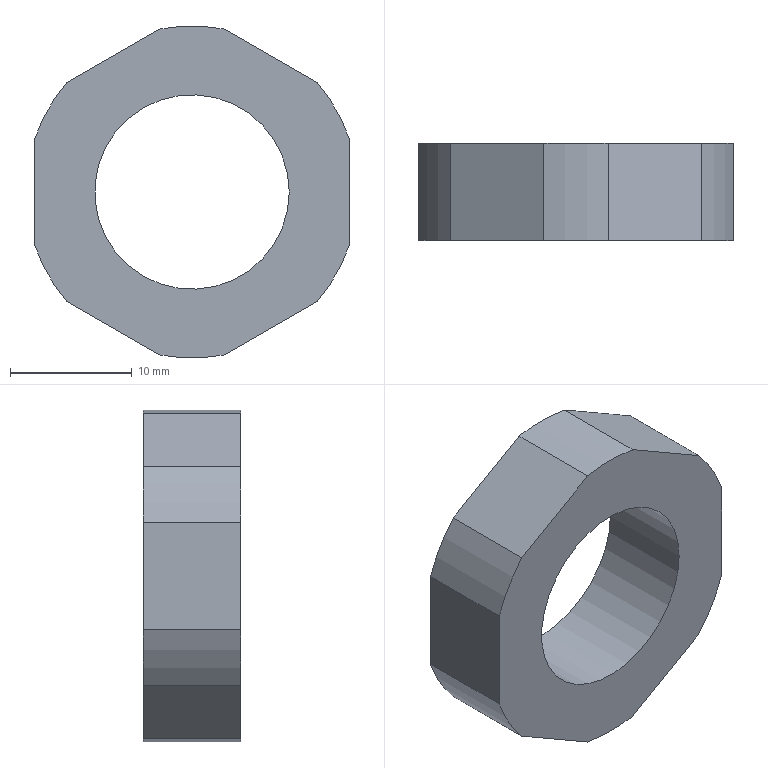Component | NX | 7 | 1 solid | 15 faces | box 25.87 x 8 x 27.34 mm | volume 2879 mm3 | plane 8 | cylinder 7 | commonest cylinder face diameters 27.34 x6 16 x1
STEP:
#1=CARTESIAN_POINT('',(0.,0.,0.));
#2=DIRECTION('',(0.,0.,1.));
#3=DIRECTION('',(1.,0.,0.));
#4=AXIS2_PLACEMENT_3D('',#1,#2,#3);
#5=CARTESIAN_POINT('',(270.398,-16.,15.578));
#6=VERTEX_POINT('',#5);
#7=CARTESIAN_POINT('',(270.398,-16.,24.422));
#8=VERTEX_POINT('',#7);
#9=CARTESIAN_POINT('',(270.398,-16.,15.578));
#10=DIRECTION('',(-0.,0.,1.));
#11=VECTOR('',#10,1.);
#12=LINE('',#9,#11);
#13=CARTESIAN_POINT('',(270.398,-8.,15.578));
#14=DIRECTION('',(1.,0.,0.));
#15=DIRECTION('',(0.,0.,-1.));
#16=AXIS2_PLACEMENT_3D('',#13,#14,#15);
#17=PLANE('',#16);
#18=CARTESIAN_POINT('',(0.,-8.));
#19=DIRECTION('',(-1.,0.));
#20=VECTOR('',#19,1.);
#21=LINE('',#18,#20);
#22=(GEOMETRIC_REPRESENTATION_CONTEXT(2)PARAMETRIC_REPRESENTATION_CONTEXT()REPRESENTATION_CONTEXT('',''));
#23=DEFINITIONAL_REPRESENTATION('',(#21),#22);
#24=PCURVE('',#17,#23);
#25=CARTESIAN_POINT('',(283.333,-16.,20.));
#26=DIRECTION('',(0.,1.,0.));
#27=DIRECTION('',(1.,0.,0.));
#28=AXIS2_PLACEMENT_3D('',#25,#26,#27);
#29=PLANE('',#28);
#30=CARTESIAN_POINT('',(-12.935,4.422));
#31=DIRECTION('',(-0.,-1.));
#32=VECTOR('',#31,1.);
#33=LINE('',#30,#32);
#34=(GEOMETRIC_REPRESENTATION_CONTEXT(2)PARAMETRIC_REPRESENTATION_CONTEXT()REPRESENTATION_CONTEXT('',''));
#35=DEFINITIONAL_REPRESENTATION('',(#33),#34);
#36=PCURVE('',#29,#35);
#37=SURFACE_CURVE('',#12,(#24,#36),.PCURVE_S1.);
#38=EDGE_CURVE('',#6,#8,#37,.T.);
#39=ORIENTED_EDGE('',*,*,#38,.T.);
#40=CARTESIAN_POINT('',(270.398,-8.,24.422));
#41=VERTEX_POINT('',#40);
#42=CARTESIAN_POINT('',(270.398,-8.,24.422));
#43=DIRECTION('',(0.,-1.,0.));
#44=VECTOR('',#43,1.);
#45=LINE('',#42,#44);
#46=CARTESIAN_POINT('',(-8.844,0.));
#47=DIRECTION('',(0.,-1.));
#48=VECTOR('',#47,1.);
#49=LINE('',#46,#48);
#50=(GEOMETRIC_REPRESENTATION_CONTEXT(2)PARAMETRIC_REPRESENTATION_CONTEXT()REPRESENTATION_CONTEXT('',''));
#51=DEFINITIONAL_REPRESENTATION('',(#49),#50);
#52=PCURVE('',#17,#51);
#53=CARTESIAN_POINT('',(283.333,-8.,20.));
#54=DIRECTION('',(0.,-1.,0.));
#55=DIRECTION('',(-1.,0.,0.));
#56=AXIS2_PLACEMENT_3D('',#53,#54,#55);
#57=CYLINDRICAL_SURFACE('',#56,13.67);
#58=CARTESIAN_POINT('',(5.954,0.));
#59=DIRECTION('',(0.,1.));
#60=VECTOR('',#59,1.);
#61=LINE('',#58,#60);
#62=(GEOMETRIC_REPRESENTATION_CONTEXT(2)PARAMETRIC_REPRESENTATION_CONTEXT()REPRESENTATION_CONTEXT('',''));
#63=DEFINITIONAL_REPRESENTATION('',(#61),#62);
#64=PCURVE('',#57,#63);
#65=SURFACE_CURVE('',#45,(#52,#64),.PCURVE_S1.);
#66=EDGE_CURVE('',#41,#8,#65,.T.);
#67=ORIENTED_EDGE('',*,*,#66,.F.);
#68=CARTESIAN_POINT('',(270.398,-8.,15.578));
#69=VERTEX_POINT('',#68);
#70=CARTESIAN_POINT('',(270.398,-8.,15.578));
#71=DIRECTION('',(-0.,0.,1.));
#72=VECTOR('',#71,1.);
#73=LINE('',#70,#72);
#74=CARTESIAN_POINT('',(0.,0.));
#75=DIRECTION('',(-1.,0.));
#76=VECTOR('',#75,1.);
#77=LINE('',#74,#76);
#78=(GEOMETRIC_REPRESENTATION_CONTEXT(2)PARAMETRIC_REPRESENTATION_CONTEXT()REPRESENTATION_CONTEXT('',''));
#79=DEFINITIONAL_REPRESENTATION('',(#77),#78);
#80=PCURVE('',#17,#79);
#81=CARTESIAN_POINT('',(283.333,-8.,20.));
#82=DIRECTION('',(0.,1.,0.));
#83=DIRECTION('',(1.,0.,0.));
#84=AXIS2_PLACEMENT_3D('',#81,#82,#83);
#85=PLANE('',#84);
#86=CARTESIAN_POINT('',(-12.935,4.422));
#87=DIRECTION('',(-0.,-1.));
#88=VECTOR('',#87,1.);
#89=LINE('',#86,#88);
#90=(GEOMETRIC_REPRESENTATION_CONTEXT(2)PARAMETRIC_REPRESENTATION_CONTEXT()REPRESENTATION_CONTEXT('',''));
#91=DEFINITIONAL_REPRESENTATION('',(#89),#90);
#92=PCURVE('',#85,#91);
#93=SURFACE_CURVE('',#73,(#80,#92),.PCURVE_S1.);
#94=EDGE_CURVE('',#69,#41,#93,.T.);
#95=ORIENTED_EDGE('',*,*,#94,.F.);
#96=CARTESIAN_POINT('',(270.398,-8.,15.578));
#97=DIRECTION('',(0.,-1.,0.));
#98=VECTOR('',#97,1.);
#99=LINE('',#96,#98);
#100=CARTESIAN_POINT('',(0.,0.));
#101=DIRECTION('',(0.,-1.));
#102=VECTOR('',#101,1.);
#103=LINE('',#100,#102);
#104=(GEOMETRIC_REPRESENTATION_CONTEXT(2)PARAMETRIC_REPRESENTATION_CONTEXT()REPRESENTATION_CONTEXT('',''));
#105=DEFINITIONAL_REPRESENTATION('',(#103),#104);
#106=PCURVE('',#17,#105);
#107=CARTESIAN_POINT('',(283.333,-8.,20.));
#108=DIRECTION('',(0.,-1.,0.));
#109=DIRECTION('',(-1.,0.,0.));
#110=AXIS2_PLACEMENT_3D('',#107,#108,#109);
#111=CYLINDRICAL_SURFACE('',#110,13.67);
#112=CARTESIAN_POINT('',(0.3294,0.));
#113=DIRECTION('',(0.,1.));
#114=VECTOR('',#113,1.);
#115=LINE('',#112,#114);
#116=(GEOMETRIC_REPRESENTATION_CONTEXT(2)PARAMETRIC_REPRESENTATION_CONTEXT()REPRESENTATION_CONTEXT('',''));
#117=DEFINITIONAL_REPRESENTATION('',(#115),#116);
#118=PCURVE('',#111,#117);
#119=SURFACE_CURVE('',#99,(#106,#118),.PCURVE_S1.);
#120=EDGE_CURVE('',#69,#6,#119,.T.);
#121=ORIENTED_EDGE('',*,*,#120,.T.);
#122=EDGE_LOOP('',(#39,#67,#95,#121));
#123=FACE_BOUND('',#122,.T.);
#124=ADVANCED_FACE('',(#123),#17,.F.);
#125=CARTESIAN_POINT('',(273.036,-16.,28.991));
#126=VERTEX_POINT('',#125);
#127=CARTESIAN_POINT('',(283.333,-16.,20.));
#128=DIRECTION('',(0.,1.,0.));
#129=DIRECTION('',(1.,0.,0.));
#130=AXIS2_PLACEMENT_3D('',#127,#128,#129);
#131=CIRCLE('',#130,13.67);
#132=CARTESIAN_POINT('',(9.425,8.));
#133=DIRECTION('',(-1.,0.));
#134=VECTOR('',#133,1.);
#135=LINE('',#132,#134);
#136=(GEOMETRIC_REPRESENTATION_CONTEXT(2)PARAMETRIC_REPRESENTATION_CONTEXT()REPRESENTATION_CONTEXT('',''));
#137=DEFINITIONAL_REPRESENTATION('',(#135),#136);
#138=PCURVE('',#57,#137);
#139=CARTESIAN_POINT('',(0.,0.));
#140=DIRECTION('',(1.,0.));
#141=AXIS2_PLACEMENT_2D('',#139,#140);
#142=CIRCLE('',#141,13.67);
#143=(GEOMETRIC_REPRESENTATION_CONTEXT(2)PARAMETRIC_REPRESENTATION_CONTEXT()REPRESENTATION_CONTEXT('',''));
#144=DEFINITIONAL_REPRESENTATION('',(#142),#143);
#145=PCURVE('',#29,#144);
#146=SURFACE_CURVE('',#131,(#138,#145),.PCURVE_S1.);
#147=EDGE_CURVE('',#8,#126,#146,.T.);
#148=ORIENTED_EDGE('',*,*,#147,.T.);
#149=CARTESIAN_POINT('',(273.036,-8.,28.991));
#150=VERTEX_POINT('',#149);
#151=CARTESIAN_POINT('',(273.036,-8.,28.991));
#152=DIRECTION('',(0.,-1.,0.));
#153=VECTOR('',#152,1.);
#154=LINE('',#151,#153);
#155=CARTESIAN_POINT('',(5.565,0.));
#156=DIRECTION('',(0.,1.));
#157=VECTOR('',#156,1.);
#158=LINE('',#155,#157);
#159=(GEOMETRIC_REPRESENTATION_CONTEXT(2)PARAMETRIC_REPRESENTATION_CONTEXT()REPRESENTATION_CONTEXT('',''));
#160=DEFINITIONAL_REPRESENTATION('',(#158),#159);
#161=PCURVE('',#57,#160);
#162=CARTESIAN_POINT('',(273.036,-8.,28.991));
#163=DIRECTION('',(0.5,0.,-0.866));
#164=DIRECTION('',(-0.866,0.,-0.5));
#165=AXIS2_PLACEMENT_3D('',#162,#163,#164);
#166=PLANE('',#165);
#167=CARTESIAN_POINT('',(-0.,0.));
#168=DIRECTION('',(0.,-1.));
#169=VECTOR('',#168,1.);
#170=LINE('',#167,#169);
#171=(GEOMETRIC_REPRESENTATION_CONTEXT(2)PARAMETRIC_REPRESENTATION_CONTEXT()REPRESENTATION_CONTEXT('',''));
#172=DEFINITIONAL_REPRESENTATION('',(#170),#171);
#173=PCURVE('',#166,#172);
#174=SURFACE_CURVE('',#154,(#161,#173),.PCURVE_S1.);
#175=EDGE_CURVE('',#150,#126,#174,.T.);
#176=ORIENTED_EDGE('',*,*,#175,.F.);
#177=CARTESIAN_POINT('',(283.333,-8.,20.));
#178=DIRECTION('',(0.,1.,0.));
#179=DIRECTION('',(1.,0.,0.));
#180=AXIS2_PLACEMENT_3D('',#177,#178,#179);
#181=CIRCLE('',#180,13.67);
#182=CARTESIAN_POINT('',(9.425,0.));
#183=DIRECTION('',(-1.,0.));
#184=VECTOR('',#183,1.);
#185=LINE('',#182,#184);
#186=(GEOMETRIC_REPRESENTATION_CONTEXT(2)PARAMETRIC_REPRESENTATION_CONTEXT()REPRESENTATION_CONTEXT('',''));
#187=DEFINITIONAL_REPRESENTATION('',(#185),#186);
#188=PCURVE('',#57,#187);
#189=CARTESIAN_POINT('',(0.,0.));
#190=DIRECTION('',(1.,0.));
#191=AXIS2_PLACEMENT_2D('',#189,#190);
#192=CIRCLE('',#191,13.67);
#193=(GEOMETRIC_REPRESENTATION_CONTEXT(2)PARAMETRIC_REPRESENTATION_CONTEXT()REPRESENTATION_CONTEXT('',''));
#194=DEFINITIONAL_REPRESENTATION('',(#192),#193);
#195=PCURVE('',#85,#194);
#196=SURFACE_CURVE('',#181,(#188,#195),.PCURVE_S1.);
#197=EDGE_CURVE('',#41,#150,#196,.T.);
#198=ORIENTED_EDGE('',*,*,#197,.F.);
#199=ORIENTED_EDGE('',*,*,#66,.T.);
#200=EDGE_LOOP('',(#148,#176,#198,#199));
#201=FACE_BOUND('',#200,.T.);
#202=ADVANCED_FACE('',(#201),#57,.T.);
#203=CARTESIAN_POINT('',(280.696,-16.,33.413));
#204=VERTEX_POINT('',#203);
#205=CARTESIAN_POINT('',(273.036,-16.,28.991));
#206=DIRECTION('',(0.866,0.,0.5));
#207=VECTOR('',#206,1.);
#208=LINE('',#205,#207);
#209=CARTESIAN_POINT('',(0.,-8.));
#210=DIRECTION('',(-1.,0.));
#211=VECTOR('',#210,1.);
#212=LINE('',#209,#211);
#213=(GEOMETRIC_REPRESENTATION_CONTEXT(2)PARAMETRIC_REPRESENTATION_CONTEXT()REPRESENTATION_CONTEXT('',''));
#214=DEFINITIONAL_REPRESENTATION('',(#212),#213);
#215=PCURVE('',#166,#214);
#216=CARTESIAN_POINT('',(-10.297,-8.991));
#217=DIRECTION('',(0.866,-0.5));
#218=VECTOR('',#217,1.);
#219=LINE('',#216,#218);
#220=(GEOMETRIC_REPRESENTATION_CONTEXT(2)PARAMETRIC_REPRESENTATION_CONTEXT()REPRESENTATION_CONTEXT('',''));
#221=DEFINITIONAL_REPRESENTATION('',(#219),#220);
#222=PCURVE('',#29,#221);
#223=SURFACE_CURVE('',#208,(#215,#222),.PCURVE_S1.);
#224=EDGE_CURVE('',#126,#204,#223,.T.);
#225=ORIENTED_EDGE('',*,*,#224,.T.);
#226=CARTESIAN_POINT('',(280.696,-8.,33.413));
#227=VERTEX_POINT('',#226);
#228=CARTESIAN_POINT('',(280.696,-8.,33.413));
#229=DIRECTION('',(0.,-1.,0.));
#230=VECTOR('',#229,1.);
#231=LINE('',#228,#230);
#232=CARTESIAN_POINT('',(-8.844,0.));
#233=DIRECTION('',(0.,-1.));
#234=VECTOR('',#233,1.);
#235=LINE('',#232,#234);
#236=(GEOMETRIC_REPRESENTATION_CONTEXT(2)PARAMETRIC_REPRESENTATION_CONTEXT()REPRESENTATION_CONTEXT('',''));
#237=DEFINITIONAL_REPRESENTATION('',(#235),#236);
#238=PCURVE('',#166,#237);
#239=CARTESIAN_POINT('',(283.333,-8.,20.));
#240=DIRECTION('',(0.,-1.,0.));
#241=DIRECTION('',(-1.,0.,0.));
#242=AXIS2_PLACEMENT_3D('',#239,#240,#241);
#243=CYLINDRICAL_SURFACE('',#242,13.67);
#244=CARTESIAN_POINT('',(4.907,0.));
#245=DIRECTION('',(0.,1.));
#246=VECTOR('',#245,1.);
#247=LINE('',#244,#246);
#248=(GEOMETRIC_REPRESENTATION_CONTEXT(2)PARAMETRIC_REPRESENTATION_CONTEXT()REPRESENTATION_CONTEXT('',''));
#249=DEFINITIONAL_REPRESENTATION('',(#247),#248);
#250=PCURVE('',#243,#249);
#251=SURFACE_CURVE('',#231,(#238,#250),.PCURVE_S1.);
#252=EDGE_CURVE('',#227,#204,#251,.T.);
#253=ORIENTED_EDGE('',*,*,#252,.F.);
#254=CARTESIAN_POINT('',(273.036,-8.,28.991));
#255=DIRECTION('',(0.866,0.,0.5));
#256=VECTOR('',#255,1.);
#257=LINE('',#254,#256);
#258=CARTESIAN_POINT('',(0.,0.));
#259=DIRECTION('',(-1.,0.));
#260=VECTOR('',#259,1.);
#261=LINE('',#258,#260);
#262=(GEOMETRIC_REPRESENTATION_CONTEXT(2)PARAMETRIC_REPRESENTATION_CONTEXT()REPRESENTATION_CONTEXT('',''));
#263=DEFINITIONAL_REPRESENTATION('',(#261),#262);
#264=PCURVE('',#166,#263);
#265=CARTESIAN_POINT('',(-10.297,-8.991));
#266=DIRECTION('',(0.866,-0.5));
#267=VECTOR('',#266,1.);
#268=LINE('',#265,#267);
#269=(GEOMETRIC_REPRESENTATION_CONTEXT(2)PARAMETRIC_REPRESENTATION_CONTEXT()REPRESENTATION_CONTEXT('',''));
#270=DEFINITIONAL_REPRESENTATION('',(#268),#269);
#271=PCURVE('',#85,#270);
#272=SURFACE_CURVE('',#257,(#264,#271),.PCURVE_S1.);
#273=EDGE_CURVE('',#150,#227,#272,.T.);
#274=ORIENTED_EDGE('',*,*,#273,.F.);
#275=ORIENTED_EDGE('',*,*,#175,.T.);
#276=EDGE_LOOP('',(#225,#253,#274,#275));
#277=FACE_BOUND('',#276,.T.);
#278=ADVANCED_FACE('',(#277),#166,.F.);
#279=CARTESIAN_POINT('',(285.971,-16.,33.413));
#280=VERTEX_POINT('',#279);
#281=CARTESIAN_POINT('',(283.333,-16.,20.));
#282=DIRECTION('',(0.,1.,0.));
#283=DIRECTION('',(1.,0.,0.));
#284=AXIS2_PLACEMENT_3D('',#281,#282,#283);
#285=CIRCLE('',#284,13.67);
#286=CARTESIAN_POINT('',(9.425,8.));
#287=DIRECTION('',(-1.,0.));
#288=VECTOR('',#287,1.);
#289=LINE('',#286,#288);
#290=(GEOMETRIC_REPRESENTATION_CONTEXT(2)PARAMETRIC_REPRESENTATION_CONTEXT()REPRESENTATION_CONTEXT('',''));
#291=DEFINITIONAL_REPRESENTATION('',(#289),#290);
#292=PCURVE('',#243,#291);
#293=CARTESIAN_POINT('',(0.,0.));
#294=DIRECTION('',(1.,0.));
#295=AXIS2_PLACEMENT_2D('',#293,#294);
#296=CIRCLE('',#295,13.67);
#297=(GEOMETRIC_REPRESENTATION_CONTEXT(2)PARAMETRIC_REPRESENTATION_CONTEXT()REPRESENTATION_CONTEXT('',''));
#298=DEFINITIONAL_REPRESENTATION('',(#296),#297);
#299=PCURVE('',#29,#298);
#300=SURFACE_CURVE('',#285,(#292,#299),.PCURVE_S1.);
#301=EDGE_CURVE('',#204,#280,#300,.T.);
#302=ORIENTED_EDGE('',*,*,#301,.T.);
#303=CARTESIAN_POINT('',(285.971,-8.,33.413));
#304=VERTEX_POINT('',#303);
#305=CARTESIAN_POINT('',(285.971,-8.,33.413));
#306=DIRECTION('',(0.,-1.,0.));
#307=VECTOR('',#306,1.);
#308=LINE('',#305,#307);
#309=CARTESIAN_POINT('',(4.518,0.));
#310=DIRECTION('',(0.,1.));
#311=VECTOR('',#310,1.);
#312=LINE('',#309,#311);
#313=(GEOMETRIC_REPRESENTATION_CONTEXT(2)PARAMETRIC_REPRESENTATION_CONTEXT()REPRESENTATION_CONTEXT('',''));
#314=DEFINITIONAL_REPRESENTATION('',(#312),#313);
#315=PCURVE('',#243,#314);
#316=CARTESIAN_POINT('',(285.971,-8.,33.413));
#317=DIRECTION('',(-0.5,0.,-0.866));
#318=DIRECTION('',(-0.866,0.,0.5));
#319=AXIS2_PLACEMENT_3D('',#316,#317,#318);
#320=PLANE('',#319);
#321=CARTESIAN_POINT('',(0.,0.));
#322=DIRECTION('',(0.,-1.));
#323=VECTOR('',#322,1.);
#324=LINE('',#321,#323);
#325=(GEOMETRIC_REPRESENTATION_CONTEXT(2)PARAMETRIC_REPRESENTATION_CONTEXT()REPRESENTATION_CONTEXT('',''));
#326=DEFINITIONAL_REPRESENTATION('',(#324),#325);
#327=PCURVE('',#320,#326);
#328=SURFACE_CURVE('',#308,(#315,#327),.PCURVE_S1.);
#329=EDGE_CURVE('',#304,#280,#328,.T.);
#330=ORIENTED_EDGE('',*,*,#329,.F.);
#331=CARTESIAN_POINT('',(283.333,-8.,20.));
#332=DIRECTION('',(0.,1.,0.));
#333=DIRECTION('',(1.,0.,0.));
#334=AXIS2_PLACEMENT_3D('',#331,#332,#333);
#335=CIRCLE('',#334,13.67);
#336=CARTESIAN_POINT('',(9.425,0.));
#337=DIRECTION('',(-1.,0.));
#338=VECTOR('',#337,1.);
#339=LINE('',#336,#338);
#340=(GEOMETRIC_REPRESENTATION_CONTEXT(2)PARAMETRIC_REPRESENTATION_CONTEXT()REPRESENTATION_CONTEXT('',''));
#341=DEFINITIONAL_REPRESENTATION('',(#339),#340);
#342=PCURVE('',#243,#341);
#343=CARTESIAN_POINT('',(0.,0.));
#344=DIRECTION('',(1.,0.));
#345=AXIS2_PLACEMENT_2D('',#343,#344);
#346=CIRCLE('',#345,13.67);
#347=(GEOMETRIC_REPRESENTATION_CONTEXT(2)PARAMETRIC_REPRESENTATION_CONTEXT()REPRESENTATION_CONTEXT('',''));
#348=DEFINITIONAL_REPRESENTATION('',(#346),#347);
#349=PCURVE('',#85,#348);
#350=SURFACE_CURVE('',#335,(#342,#349),.PCURVE_S1.);
#351=EDGE_CURVE('',#227,#304,#350,.T.);
#352=ORIENTED_EDGE('',*,*,#351,.F.);
#353=ORIENTED_EDGE('',*,*,#252,.T.);
#354=EDGE_LOOP('',(#302,#330,#352,#353));
#355=FACE_BOUND('',#354,.T.);
#356=ADVANCED_FACE('',(#355),#243,.T.);
#357=CARTESIAN_POINT('',(293.631,-16.,28.991));
#358=VERTEX_POINT('',#357);
#359=CARTESIAN_POINT('',(285.971,-16.,33.413));
#360=DIRECTION('',(0.866,0.,-0.5));
#361=VECTOR('',#360,1.);
#362=LINE('',#359,#361);
#363=CARTESIAN_POINT('',(0.,-8.));
#364=DIRECTION('',(-1.,0.));
#365=VECTOR('',#364,1.);
#366=LINE('',#363,#365);
#367=(GEOMETRIC_REPRESENTATION_CONTEXT(2)PARAMETRIC_REPRESENTATION_CONTEXT()REPRESENTATION_CONTEXT('',''));
#368=DEFINITIONAL_REPRESENTATION('',(#366),#367);
#369=PCURVE('',#320,#368);
#370=CARTESIAN_POINT('',(2.638,-13.413));
#371=DIRECTION('',(0.866,0.5));
#372=VECTOR('',#371,1.);
#373=LINE('',#370,#372);
#374=(GEOMETRIC_REPRESENTATION_CONTEXT(2)PARAMETRIC_REPRESENTATION_CONTEXT()REPRESENTATION_CONTEXT('',''));
#375=DEFINITIONAL_REPRESENTATION('',(#373),#374);
#376=PCURVE('',#29,#375);
#377=SURFACE_CURVE('',#362,(#369,#376),.PCURVE_S1.);
#378=EDGE_CURVE('',#280,#358,#377,.T.);
#379=ORIENTED_EDGE('',*,*,#378,.T.);
#380=CARTESIAN_POINT('',(293.631,-8.,28.991));
#381=VERTEX_POINT('',#380);
#382=CARTESIAN_POINT('',(293.631,-8.,28.991));
#383=DIRECTION('',(0.,-1.,0.));
#384=VECTOR('',#383,1.);
#385=LINE('',#382,#384);
#386=CARTESIAN_POINT('',(-8.844,0.));
#387=DIRECTION('',(0.,-1.));
#388=VECTOR('',#387,1.);
#389=LINE('',#386,#388);
#390=(GEOMETRIC_REPRESENTATION_CONTEXT(2)PARAMETRIC_REPRESENTATION_CONTEXT()REPRESENTATION_CONTEXT('',''));
#391=DEFINITIONAL_REPRESENTATION('',(#389),#390);
#392=PCURVE('',#320,#391);
#393=CARTESIAN_POINT('',(283.333,-8.,20.));
#394=DIRECTION('',(0.,-1.,0.));
#395=DIRECTION('',(-1.,0.,0.));
#396=AXIS2_PLACEMENT_3D('',#393,#394,#395);
#397=CYLINDRICAL_SURFACE('',#396,13.67);
#398=CARTESIAN_POINT('',(3.859,0.));
#399=DIRECTION('',(0.,1.));
#400=VECTOR('',#399,1.);
#401=LINE('',#398,#400);
#402=(GEOMETRIC_REPRESENTATION_CONTEXT(2)PARAMETRIC_REPRESENTATION_CONTEXT()REPRESENTATION_CONTEXT('',''));
#403=DEFINITIONAL_REPRESENTATION('',(#401),#402);
#404=PCURVE('',#397,#403);
#405=SURFACE_CURVE('',#385,(#392,#404),.PCURVE_S1.);
#406=EDGE_CURVE('',#381,#358,#405,.T.);
#407=ORIENTED_EDGE('',*,*,#406,.F.);
#408=CARTESIAN_POINT('',(285.971,-8.,33.413));
#409=DIRECTION('',(0.866,0.,-0.5));
#410=VECTOR('',#409,1.);
#411=LINE('',#408,#410);
#412=CARTESIAN_POINT('',(0.,0.));
#413=DIRECTION('',(-1.,0.));
#414=VECTOR('',#413,1.);
#415=LINE('',#412,#414);
#416=(GEOMETRIC_REPRESENTATION_CONTEXT(2)PARAMETRIC_REPRESENTATION_CONTEXT()REPRESENTATION_CONTEXT('',''));
#417=DEFINITIONAL_REPRESENTATION('',(#415),#416);
#418=PCURVE('',#320,#417);
#419=CARTESIAN_POINT('',(2.638,-13.413));
#420=DIRECTION('',(0.866,0.5));
#421=VECTOR('',#420,1.);
#422=LINE('',#419,#421);
#423=(GEOMETRIC_REPRESENTATION_CONTEXT(2)PARAMETRIC_REPRESENTATION_CONTEXT()REPRESENTATION_CONTEXT('',''));
#424=DEFINITIONAL_REPRESENTATION('',(#422),#423);
#425=PCURVE('',#85,#424);
#426=SURFACE_CURVE('',#411,(#418,#425),.PCURVE_S1.);
#427=EDGE_CURVE('',#304,#381,#426,.T.);
#428=ORIENTED_EDGE('',*,*,#427,.F.);
#429=ORIENTED_EDGE('',*,*,#329,.T.);
#430=EDGE_LOOP('',(#379,#407,#428,#429));
#431=FACE_BOUND('',#430,.T.);
#432=ADVANCED_FACE('',(#431),#320,.F.);
#433=CARTESIAN_POINT('',(296.268,-16.,24.422));
#434=VERTEX_POINT('',#433);
#435=CARTESIAN_POINT('',(283.333,-16.,20.));
#436=DIRECTION('',(0.,1.,0.));
#437=DIRECTION('',(1.,0.,0.));
#438=AXIS2_PLACEMENT_3D('',#435,#436,#437);
#439=CIRCLE('',#438,13.67);
#440=CARTESIAN_POINT('',(9.425,8.));
#441=DIRECTION('',(-1.,0.));
#442=VECTOR('',#441,1.);
#443=LINE('',#440,#442);
#444=(GEOMETRIC_REPRESENTATION_CONTEXT(2)PARAMETRIC_REPRESENTATION_CONTEXT()REPRESENTATION_CONTEXT('',''));
#445=DEFINITIONAL_REPRESENTATION('',(#443),#444);
#446=PCURVE('',#397,#445);
#447=CARTESIAN_POINT('',(0.,0.));
#448=DIRECTION('',(1.,0.));
#449=AXIS2_PLACEMENT_2D('',#447,#448);
#450=CIRCLE('',#449,13.67);
#451=(GEOMETRIC_REPRESENTATION_CONTEXT(2)PARAMETRIC_REPRESENTATION_CONTEXT()REPRESENTATION_CONTEXT('',''));
#452=DEFINITIONAL_REPRESENTATION('',(#450),#451);
#453=PCURVE('',#29,#452);
#454=SURFACE_CURVE('',#439,(#446,#453),.PCURVE_S1.);
#455=EDGE_CURVE('',#358,#434,#454,.T.);
#456=ORIENTED_EDGE('',*,*,#455,.T.);
#457=CARTESIAN_POINT('',(296.268,-8.,24.422));
#458=VERTEX_POINT('',#457);
#459=CARTESIAN_POINT('',(296.268,-8.,24.422));
#460=DIRECTION('',(0.,-1.,0.));
#461=VECTOR('',#460,1.);
#462=LINE('',#459,#461);
#463=CARTESIAN_POINT('',(3.471,0.));
#464=DIRECTION('',(0.,1.));
#465=VECTOR('',#464,1.);
#466=LINE('',#463,#465);
#467=(GEOMETRIC_REPRESENTATION_CONTEXT(2)PARAMETRIC_REPRESENTATION_CONTEXT()REPRESENTATION_CONTEXT('',''));
#468=DEFINITIONAL_REPRESENTATION('',(#466),#467);
#469=PCURVE('',#397,#468);
#470=CARTESIAN_POINT('',(296.268,-8.,24.422));
#471=DIRECTION('',(-1.,0.,-0.));
#472=DIRECTION('',(-0.,0.,1.));
#473=AXIS2_PLACEMENT_3D('',#470,#471,#472);
#474=PLANE('',#473);
#475=CARTESIAN_POINT('',(-0.,0.));
#476=DIRECTION('',(0.,-1.));
#477=VECTOR('',#476,1.);
#478=LINE('',#475,#477);
#479=(GEOMETRIC_REPRESENTATION_CONTEXT(2)PARAMETRIC_REPRESENTATION_CONTEXT()REPRESENTATION_CONTEXT('',''));
#480=DEFINITIONAL_REPRESENTATION('',(#478),#479);
#481=PCURVE('',#474,#480);
#482=SURFACE_CURVE('',#462,(#469,#481),.PCURVE_S1.);
#483=EDGE_CURVE('',#458,#434,#482,.T.);
#484=ORIENTED_EDGE('',*,*,#483,.F.);
#485=CARTESIAN_POINT('',(283.333,-8.,20.));
#486=DIRECTION('',(0.,1.,0.));
#487=DIRECTION('',(1.,0.,0.));
#488=AXIS2_PLACEMENT_3D('',#485,#486,#487);
#489=CIRCLE('',#488,13.67);
#490=CARTESIAN_POINT('',(9.425,0.));
#491=DIRECTION('',(-1.,0.));
#492=VECTOR('',#491,1.);
#493=LINE('',#490,#492);
#494=(GEOMETRIC_REPRESENTATION_CONTEXT(2)PARAMETRIC_REPRESENTATION_CONTEXT()REPRESENTATION_CONTEXT('',''));
#495=DEFINITIONAL_REPRESENTATION('',(#493),#494);
#496=PCURVE('',#397,#495);
#497=CARTESIAN_POINT('',(0.,0.));
#498=DIRECTION('',(1.,0.));
#499=AXIS2_PLACEMENT_2D('',#497,#498);
#500=CIRCLE('',#499,13.67);
#501=(GEOMETRIC_REPRESENTATION_CONTEXT(2)PARAMETRIC_REPRESENTATION_CONTEXT()REPRESENTATION_CONTEXT('',''));
#502=DEFINITIONAL_REPRESENTATION('',(#500),#501);
#503=PCURVE('',#85,#502);
#504=SURFACE_CURVE('',#489,(#496,#503),.PCURVE_S1.);
#505=EDGE_CURVE('',#381,#458,#504,.T.);
#506=ORIENTED_EDGE('',*,*,#505,.F.);
#507=ORIENTED_EDGE('',*,*,#406,.T.);
#508=EDGE_LOOP('',(#456,#484,#506,#507));
#509=FACE_BOUND('',#508,.T.);
#510=ADVANCED_FACE('',(#509),#397,.T.);
#511=CARTESIAN_POINT('',(296.268,-16.,15.578));
#512=VERTEX_POINT('',#511);
#513=CARTESIAN_POINT('',(296.268,-16.,24.422));
#514=DIRECTION('',(0.,0.,-1.));
#515=VECTOR('',#514,1.);
#516=LINE('',#513,#515);
#517=CARTESIAN_POINT('',(0.,-8.));
#518=DIRECTION('',(-1.,0.));
#519=VECTOR('',#518,1.);
#520=LINE('',#517,#519);
#521=(GEOMETRIC_REPRESENTATION_CONTEXT(2)PARAMETRIC_REPRESENTATION_CONTEXT()REPRESENTATION_CONTEXT('',''));
#522=DEFINITIONAL_REPRESENTATION('',(#520),#521);
#523=PCURVE('',#474,#522);
#524=CARTESIAN_POINT('',(12.935,-4.422));
#525=DIRECTION('',(0.,1.));
#526=VECTOR('',#525,1.);
#527=LINE('',#524,#526);
#528=(GEOMETRIC_REPRESENTATION_CONTEXT(2)PARAMETRIC_REPRESENTATION_CONTEXT()REPRESENTATION_CONTEXT('',''));
#529=DEFINITIONAL_REPRESENTATION('',(#527),#528);
#530=PCURVE('',#29,#529);
#531=SURFACE_CURVE('',#516,(#523,#530),.PCURVE_S1.);
#532=EDGE_CURVE('',#434,#512,#531,.T.);
#533=ORIENTED_EDGE('',*,*,#532,.T.);
#534=CARTESIAN_POINT('',(296.268,-8.,15.578));
#535=VERTEX_POINT('',#534);
#536=CARTESIAN_POINT('',(296.268,-8.,15.578));
#537=DIRECTION('',(0.,-1.,0.));
#538=VECTOR('',#537,1.);
#539=LINE('',#536,#538);
#540=CARTESIAN_POINT('',(-8.844,0.));
#541=DIRECTION('',(0.,-1.));
#542=VECTOR('',#541,1.);
#543=LINE('',#540,#542);
#544=(GEOMETRIC_REPRESENTATION_CONTEXT(2)PARAMETRIC_REPRESENTATION_CONTEXT()REPRESENTATION_CONTEXT('',''));
#545=DEFINITIONAL_REPRESENTATION('',(#543),#544);
#546=PCURVE('',#474,#545);
#547=CARTESIAN_POINT('',(283.333,-8.,20.));
#548=DIRECTION('',(0.,-1.,0.));
#549=DIRECTION('',(-1.,0.,0.));
#550=AXIS2_PLACEMENT_3D('',#547,#548,#549);
#551=CYLINDRICAL_SURFACE('',#550,13.67);
#552=CARTESIAN_POINT('',(2.812,0.));
#553=DIRECTION('',(0.,1.));
#554=VECTOR('',#553,1.);
#555=LINE('',#552,#554);
#556=(GEOMETRIC_REPRESENTATION_CONTEXT(2)PARAMETRIC_REPRESENTATION_CONTEXT()REPRESENTATION_CONTEXT('',''));
#557=DEFINITIONAL_REPRESENTATION('',(#555),#556);
#558=PCURVE('',#551,#557);
#559=SURFACE_CURVE('',#539,(#546,#558),.PCURVE_S1.);
#560=EDGE_CURVE('',#535,#512,#559,.T.);
#561=ORIENTED_EDGE('',*,*,#560,.F.);
#562=CARTESIAN_POINT('',(296.268,-8.,24.422));
#563=DIRECTION('',(0.,0.,-1.));
#564=VECTOR('',#563,1.);
#565=LINE('',#562,#564);
#566=CARTESIAN_POINT('',(0.,0.));
#567=DIRECTION('',(-1.,0.));
#568=VECTOR('',#567,1.);
#569=LINE('',#566,#568);
#570=(GEOMETRIC_REPRESENTATION_CONTEXT(2)PARAMETRIC_REPRESENTATION_CONTEXT()REPRESENTATION_CONTEXT('',''));
#571=DEFINITIONAL_REPRESENTATION('',(#569),#570);
#572=PCURVE('',#474,#571);
#573=CARTESIAN_POINT('',(12.935,-4.422));
#574=DIRECTION('',(0.,1.));
#575=VECTOR('',#574,1.);
#576=LINE('',#573,#575);
#577=(GEOMETRIC_REPRESENTATION_CONTEXT(2)PARAMETRIC_REPRESENTATION_CONTEXT()REPRESENTATION_CONTEXT('',''));
#578=DEFINITIONAL_REPRESENTATION('',(#576),#577);
#579=PCURVE('',#85,#578);
#580=SURFACE_CURVE('',#565,(#572,#579),.PCURVE_S1.);
#581=EDGE_CURVE('',#458,#535,#580,.T.);
#582=ORIENTED_EDGE('',*,*,#581,.F.);
#583=ORIENTED_EDGE('',*,*,#483,.T.);
#584=EDGE_LOOP('',(#533,#561,#582,#583));
#585=FACE_BOUND('',#584,.T.);
#586=ADVANCED_FACE('',(#585),#474,.F.);
#587=CARTESIAN_POINT('',(293.631,-16.,11.009));
#588=VERTEX_POINT('',#587);
#589=CARTESIAN_POINT('',(283.333,-16.,20.));
#590=DIRECTION('',(0.,1.,0.));
#591=DIRECTION('',(1.,0.,0.));
#592=AXIS2_PLACEMENT_3D('',#589,#590,#591);
#593=CIRCLE('',#592,13.67);
#594=CARTESIAN_POINT('',(3.142,8.));
#595=DIRECTION('',(-1.,0.));
#596=VECTOR('',#595,1.);
#597=LINE('',#594,#596);
#598=(GEOMETRIC_REPRESENTATION_CONTEXT(2)PARAMETRIC_REPRESENTATION_CONTEXT()REPRESENTATION_CONTEXT('',''));
#599=DEFINITIONAL_REPRESENTATION('',(#597),#598);
#600=PCURVE('',#551,#599);
#601=CARTESIAN_POINT('',(0.,0.));
#602=DIRECTION('',(1.,0.));
#603=AXIS2_PLACEMENT_2D('',#601,#602);
#604=CIRCLE('',#603,13.67);
#605=(GEOMETRIC_REPRESENTATION_CONTEXT(2)PARAMETRIC_REPRESENTATION_CONTEXT()REPRESENTATION_CONTEXT('',''));
#606=DEFINITIONAL_REPRESENTATION('',(#604),#605);
#607=PCURVE('',#29,#606);
#608=SURFACE_CURVE('',#593,(#600,#607),.PCURVE_S1.);
#609=EDGE_CURVE('',#512,#588,#608,.T.);
#610=ORIENTED_EDGE('',*,*,#609,.T.);
#611=CARTESIAN_POINT('',(293.631,-8.,11.009));
#612=VERTEX_POINT('',#611);
#613=CARTESIAN_POINT('',(293.631,-8.,11.009));
#614=DIRECTION('',(0.,-1.,0.));
#615=VECTOR('',#614,1.);
#616=LINE('',#613,#615);
#617=CARTESIAN_POINT('',(2.424,0.));
#618=DIRECTION('',(0.,1.));
#619=VECTOR('',#618,1.);
#620=LINE('',#617,#619);
#621=(GEOMETRIC_REPRESENTATION_CONTEXT(2)PARAMETRIC_REPRESENTATION_CONTEXT()REPRESENTATION_CONTEXT('',''));
#622=DEFINITIONAL_REPRESENTATION('',(#620),#621);
#623=PCURVE('',#551,#622);
#624=CARTESIAN_POINT('',(293.631,-8.,11.009));
#625=DIRECTION('',(-0.5,0.,0.866));
#626=DIRECTION('',(0.866,0.,0.5));
#627=AXIS2_PLACEMENT_3D('',#624,#625,#626);
#628=PLANE('',#627);
#629=CARTESIAN_POINT('',(-0.,0.));
#630=DIRECTION('',(0.,-1.));
#631=VECTOR('',#630,1.);
#632=LINE('',#629,#631);
#633=(GEOMETRIC_REPRESENTATION_CONTEXT(2)PARAMETRIC_REPRESENTATION_CONTEXT()REPRESENTATION_CONTEXT('',''));
#634=DEFINITIONAL_REPRESENTATION('',(#632),#633);
#635=PCURVE('',#628,#634);
#636=SURFACE_CURVE('',#616,(#623,#635),.PCURVE_S1.);
#637=EDGE_CURVE('',#612,#588,#636,.T.);
#638=ORIENTED_EDGE('',*,*,#637,.F.);
#639=CARTESIAN_POINT('',(283.333,-8.,20.));
#640=DIRECTION('',(0.,1.,0.));
#641=DIRECTION('',(1.,0.,0.));
#642=AXIS2_PLACEMENT_3D('',#639,#640,#641);
#643=CIRCLE('',#642,13.67);
#644=CARTESIAN_POINT('',(3.142,0.));
#645=DIRECTION('',(-1.,0.));
#646=VECTOR('',#645,1.);
#647=LINE('',#644,#646);
#648=(GEOMETRIC_REPRESENTATION_CONTEXT(2)PARAMETRIC_REPRESENTATION_CONTEXT()REPRESENTATION_CONTEXT('',''));
#649=DEFINITIONAL_REPRESENTATION('',(#647),#648);
#650=PCURVE('',#551,#649);
#651=CARTESIAN_POINT('',(0.,0.));
#652=DIRECTION('',(1.,0.));
#653=AXIS2_PLACEMENT_2D('',#651,#652);
#654=CIRCLE('',#653,13.67);
#655=(GEOMETRIC_REPRESENTATION_CONTEXT(2)PARAMETRIC_REPRESENTATION_CONTEXT()REPRESENTATION_CONTEXT('',''));
#656=DEFINITIONAL_REPRESENTATION('',(#654),#655);
#657=PCURVE('',#85,#656);
#658=SURFACE_CURVE('',#643,(#650,#657),.PCURVE_S1.);
#659=EDGE_CURVE('',#535,#612,#658,.T.);
#660=ORIENTED_EDGE('',*,*,#659,.F.);
#661=ORIENTED_EDGE('',*,*,#560,.T.);
#662=EDGE_LOOP('',(#610,#638,#660,#661));
#663=FACE_BOUND('',#662,.T.);
#664=ADVANCED_FACE('',(#663),#551,.T.);
#665=CARTESIAN_POINT('',(285.971,-16.,6.587));
#666=VERTEX_POINT('',#665);
#667=CARTESIAN_POINT('',(293.631,-16.,11.009));
#668=DIRECTION('',(-0.866,0.,-0.5));
#669=VECTOR('',#668,1.);
#670=LINE('',#667,#669);
#671=CARTESIAN_POINT('',(0.,-8.));
#672=DIRECTION('',(-1.,0.));
#673=VECTOR('',#672,1.);
#674=LINE('',#671,#673);
#675=(GEOMETRIC_REPRESENTATION_CONTEXT(2)PARAMETRIC_REPRESENTATION_CONTEXT()REPRESENTATION_CONTEXT('',''));
#676=DEFINITIONAL_REPRESENTATION('',(#674),#675);
#677=PCURVE('',#628,#676);
#678=CARTESIAN_POINT('',(10.297,8.991));
#679=DIRECTION('',(-0.866,0.5));
#680=VECTOR('',#679,1.);
#681=LINE('',#678,#680);
#682=(GEOMETRIC_REPRESENTATION_CONTEXT(2)PARAMETRIC_REPRESENTATION_CONTEXT()REPRESENTATION_CONTEXT('',''));
#683=DEFINITIONAL_REPRESENTATION('',(#681),#682);
#684=PCURVE('',#29,#683);
#685=SURFACE_CURVE('',#670,(#677,#684),.PCURVE_S1.);
#686=EDGE_CURVE('',#588,#666,#685,.T.);
#687=ORIENTED_EDGE('',*,*,#686,.T.);
#688=CARTESIAN_POINT('',(285.971,-8.,6.587));
#689=VERTEX_POINT('',#688);
#690=CARTESIAN_POINT('',(285.971,-8.,6.587));
#691=DIRECTION('',(0.,-1.,0.));
#692=VECTOR('',#691,1.);
#693=LINE('',#690,#692);
#694=CARTESIAN_POINT('',(-8.844,0.));
#695=DIRECTION('',(0.,-1.));
#696=VECTOR('',#695,1.);
#697=LINE('',#694,#696);
#698=(GEOMETRIC_REPRESENTATION_CONTEXT(2)PARAMETRIC_REPRESENTATION_CONTEXT()REPRESENTATION_CONTEXT('',''));
#699=DEFINITIONAL_REPRESENTATION('',(#697),#698);
#700=PCURVE('',#628,#699);
#701=CARTESIAN_POINT('',(283.333,-8.,20.));
#702=DIRECTION('',(0.,-1.,0.));
#703=DIRECTION('',(-1.,0.,0.));
#704=AXIS2_PLACEMENT_3D('',#701,#702,#703);
#705=CYLINDRICAL_SURFACE('',#704,13.67);
#706=CARTESIAN_POINT('',(1.765,0.));
#707=DIRECTION('',(0.,1.));
#708=VECTOR('',#707,1.);
#709=LINE('',#706,#708);
#710=(GEOMETRIC_REPRESENTATION_CONTEXT(2)PARAMETRIC_REPRESENTATION_CONTEXT()REPRESENTATION_CONTEXT('',''));
#711=DEFINITIONAL_REPRESENTATION('',(#709),#710);
#712=PCURVE('',#705,#711);
#713=SURFACE_CURVE('',#693,(#700,#712),.PCURVE_S1.);
#714=EDGE_CURVE('',#689,#666,#713,.T.);
#715=ORIENTED_EDGE('',*,*,#714,.F.);
#716=CARTESIAN_POINT('',(293.631,-8.,11.009));
#717=DIRECTION('',(-0.866,0.,-0.5));
#718=VECTOR('',#717,1.);
#719=LINE('',#716,#718);
#720=CARTESIAN_POINT('',(0.,0.));
#721=DIRECTION('',(-1.,0.));
#722=VECTOR('',#721,1.);
#723=LINE('',#720,#722);
#724=(GEOMETRIC_REPRESENTATION_CONTEXT(2)PARAMETRIC_REPRESENTATION_CONTEXT()REPRESENTATION_CONTEXT('',''));
#725=DEFINITIONAL_REPRESENTATION('',(#723),#724);
#726=PCURVE('',#628,#725);
#727=CARTESIAN_POINT('',(10.297,8.991));
#728=DIRECTION('',(-0.866,0.5));
#729=VECTOR('',#728,1.);
#730=LINE('',#727,#729);
#731=(GEOMETRIC_REPRESENTATION_CONTEXT(2)PARAMETRIC_REPRESENTATION_CONTEXT()REPRESENTATION_CONTEXT('',''));
#732=DEFINITIONAL_REPRESENTATION('',(#730),#731);
#733=PCURVE('',#85,#732);
#734=SURFACE_CURVE('',#719,(#726,#733),.PCURVE_S1.);
#735=EDGE_CURVE('',#612,#689,#734,.T.);
#736=ORIENTED_EDGE('',*,*,#735,.F.);
#737=ORIENTED_EDGE('',*,*,#637,.T.);
#738=EDGE_LOOP('',(#687,#715,#736,#737));
#739=FACE_BOUND('',#738,.T.);
#740=ADVANCED_FACE('',(#739),#628,.F.);
#741=CARTESIAN_POINT('',(280.696,-16.,6.587));
#742=VERTEX_POINT('',#741);
#743=CARTESIAN_POINT('',(283.333,-16.,20.));
#744=DIRECTION('',(0.,1.,0.));
#745=DIRECTION('',(1.,0.,0.));
#746=AXIS2_PLACEMENT_3D('',#743,#744,#745);
#747=CIRCLE('',#746,13.67);
#748=CARTESIAN_POINT('',(3.142,8.));
#749=DIRECTION('',(-1.,0.));
#750=VECTOR('',#749,1.);
#751=LINE('',#748,#750);
#752=(GEOMETRIC_REPRESENTATION_CONTEXT(2)PARAMETRIC_REPRESENTATION_CONTEXT()REPRESENTATION_CONTEXT('',''));
#753=DEFINITIONAL_REPRESENTATION('',(#751),#752);
#754=PCURVE('',#705,#753);
#755=CARTESIAN_POINT('',(0.,0.));
#756=DIRECTION('',(1.,0.));
#757=AXIS2_PLACEMENT_2D('',#755,#756);
#758=CIRCLE('',#757,13.67);
#759=(GEOMETRIC_REPRESENTATION_CONTEXT(2)PARAMETRIC_REPRESENTATION_CONTEXT()REPRESENTATION_CONTEXT('',''));
#760=DEFINITIONAL_REPRESENTATION('',(#758),#759);
#761=PCURVE('',#29,#760);
#762=SURFACE_CURVE('',#747,(#754,#761),.PCURVE_S1.);
#763=EDGE_CURVE('',#666,#742,#762,.T.);
#764=ORIENTED_EDGE('',*,*,#763,.T.);
#765=CARTESIAN_POINT('',(280.696,-8.,6.587));
#766=VERTEX_POINT('',#765);
#767=CARTESIAN_POINT('',(280.696,-8.,6.587));
#768=DIRECTION('',(0.,-1.,0.));
#769=VECTOR('',#768,1.);
#770=LINE('',#767,#769);
#771=CARTESIAN_POINT('',(1.377,0.));
#772=DIRECTION('',(0.,1.));
#773=VECTOR('',#772,1.);
#774=LINE('',#771,#773);
#775=(GEOMETRIC_REPRESENTATION_CONTEXT(2)PARAMETRIC_REPRESENTATION_CONTEXT()REPRESENTATION_CONTEXT('',''));
#776=DEFINITIONAL_REPRESENTATION('',(#774),#775);
#777=PCURVE('',#705,#776);
#778=CARTESIAN_POINT('',(280.696,-8.,6.587));
#779=DIRECTION('',(0.5,0.,0.866));
#780=DIRECTION('',(0.866,0.,-0.5));
#781=AXIS2_PLACEMENT_3D('',#778,#779,#780);
#782=PLANE('',#781);
#783=CARTESIAN_POINT('',(-0.,0.));
#784=DIRECTION('',(0.,-1.));
#785=VECTOR('',#784,1.);
#786=LINE('',#783,#785);
#787=(GEOMETRIC_REPRESENTATION_CONTEXT(2)PARAMETRIC_REPRESENTATION_CONTEXT()REPRESENTATION_CONTEXT('',''));
#788=DEFINITIONAL_REPRESENTATION('',(#786),#787);
#789=PCURVE('',#782,#788);
#790=SURFACE_CURVE('',#770,(#777,#789),.PCURVE_S1.);
#791=EDGE_CURVE('',#766,#742,#790,.T.);
#792=ORIENTED_EDGE('',*,*,#791,.F.);
#793=CARTESIAN_POINT('',(283.333,-8.,20.));
#794=DIRECTION('',(0.,1.,0.));
#795=DIRECTION('',(1.,0.,0.));
#796=AXIS2_PLACEMENT_3D('',#793,#794,#795);
#797=CIRCLE('',#796,13.67);
#798=CARTESIAN_POINT('',(3.142,0.));
#799=DIRECTION('',(-1.,0.));
#800=VECTOR('',#799,1.);
#801=LINE('',#798,#800);
#802=(GEOMETRIC_REPRESENTATION_CONTEXT(2)PARAMETRIC_REPRESENTATION_CONTEXT()REPRESENTATION_CONTEXT('',''));
#803=DEFINITIONAL_REPRESENTATION('',(#801),#802);
#804=PCURVE('',#705,#803);
#805=CARTESIAN_POINT('',(0.,0.));
#806=DIRECTION('',(1.,0.));
#807=AXIS2_PLACEMENT_2D('',#805,#806);
#808=CIRCLE('',#807,13.67);
#809=(GEOMETRIC_REPRESENTATION_CONTEXT(2)PARAMETRIC_REPRESENTATION_CONTEXT()REPRESENTATION_CONTEXT('',''));
#810=DEFINITIONAL_REPRESENTATION('',(#808),#809);
#811=PCURVE('',#85,#810);
#812=SURFACE_CURVE('',#797,(#804,#811),.PCURVE_S1.);
#813=EDGE_CURVE('',#689,#766,#812,.T.);
#814=ORIENTED_EDGE('',*,*,#813,.F.);
#815=ORIENTED_EDGE('',*,*,#714,.T.);
#816=EDGE_LOOP('',(#764,#792,#814,#815));
#817=FACE_BOUND('',#816,.T.);
#818=ADVANCED_FACE('',(#817),#705,.T.);
#819=CARTESIAN_POINT('',(273.036,-16.,11.009));
#820=VERTEX_POINT('',#819);
#821=CARTESIAN_POINT('',(280.696,-16.,6.587));
#822=DIRECTION('',(-0.866,0.,0.5));
#823=VECTOR('',#822,1.);
#824=LINE('',#821,#823);
#825=CARTESIAN_POINT('',(0.,-8.));
#826=DIRECTION('',(-1.,0.));
#827=VECTOR('',#826,1.);
#828=LINE('',#825,#827);
#829=(GEOMETRIC_REPRESENTATION_CONTEXT(2)PARAMETRIC_REPRESENTATION_CONTEXT()REPRESENTATION_CONTEXT('',''));
#830=DEFINITIONAL_REPRESENTATION('',(#828),#829);
#831=PCURVE('',#782,#830);
#832=CARTESIAN_POINT('',(-2.638,13.413));
#833=DIRECTION('',(-0.866,-0.5));
#834=VECTOR('',#833,1.);
#835=LINE('',#832,#834);
#836=(GEOMETRIC_REPRESENTATION_CONTEXT(2)PARAMETRIC_REPRESENTATION_CONTEXT()REPRESENTATION_CONTEXT('',''));
#837=DEFINITIONAL_REPRESENTATION('',(#835),#836);
#838=PCURVE('',#29,#837);
#839=SURFACE_CURVE('',#824,(#831,#838),.PCURVE_S1.);
#840=EDGE_CURVE('',#742,#820,#839,.T.);
#841=ORIENTED_EDGE('',*,*,#840,.T.);
#842=CARTESIAN_POINT('',(273.036,-8.,11.009));
#843=VERTEX_POINT('',#842);
#844=CARTESIAN_POINT('',(273.036,-8.,11.009));
#845=DIRECTION('',(0.,-1.,0.));
#846=VECTOR('',#845,1.);
#847=LINE('',#844,#846);
#848=CARTESIAN_POINT('',(-8.844,0.));
#849=DIRECTION('',(0.,-1.));
#850=VECTOR('',#849,1.);
#851=LINE('',#848,#850);
#852=(GEOMETRIC_REPRESENTATION_CONTEXT(2)PARAMETRIC_REPRESENTATION_CONTEXT()REPRESENTATION_CONTEXT('',''));
#853=DEFINITIONAL_REPRESENTATION('',(#851),#852);
#854=PCURVE('',#782,#853);
#855=CARTESIAN_POINT('',(0.7178,0.));
#856=DIRECTION('',(0.,1.));
#857=VECTOR('',#856,1.);
#858=LINE('',#855,#857);
#859=(GEOMETRIC_REPRESENTATION_CONTEXT(2)PARAMETRIC_REPRESENTATION_CONTEXT()REPRESENTATION_CONTEXT('',''));
#860=DEFINITIONAL_REPRESENTATION('',(#858),#859);
#861=PCURVE('',#111,#860);
#862=SURFACE_CURVE('',#847,(#854,#861),.PCURVE_S1.);
#863=EDGE_CURVE('',#843,#820,#862,.T.);
#864=ORIENTED_EDGE('',*,*,#863,.F.);
#865=CARTESIAN_POINT('',(280.696,-8.,6.587));
#866=DIRECTION('',(-0.866,0.,0.5));
#867=VECTOR('',#866,1.);
#868=LINE('',#865,#867);
#869=CARTESIAN_POINT('',(0.,0.));
#870=DIRECTION('',(-1.,0.));
#871=VECTOR('',#870,1.);
#872=LINE('',#869,#871);
#873=(GEOMETRIC_REPRESENTATION_CONTEXT(2)PARAMETRIC_REPRESENTATION_CONTEXT()REPRESENTATION_CONTEXT('',''));
#874=DEFINITIONAL_REPRESENTATION('',(#872),#873);
#875=PCURVE('',#782,#874);
#876=CARTESIAN_POINT('',(-2.638,13.413));
#877=DIRECTION('',(-0.866,-0.5));
#878=VECTOR('',#877,1.);
#879=LINE('',#876,#878);
#880=(GEOMETRIC_REPRESENTATION_CONTEXT(2)PARAMETRIC_REPRESENTATION_CONTEXT()REPRESENTATION_CONTEXT('',''));
#881=DEFINITIONAL_REPRESENTATION('',(#879),#880);
#882=PCURVE('',#85,#881);
#883=SURFACE_CURVE('',#868,(#875,#882),.PCURVE_S1.);
#884=EDGE_CURVE('',#766,#843,#883,.T.);
#885=ORIENTED_EDGE('',*,*,#884,.F.);
#886=ORIENTED_EDGE('',*,*,#791,.T.);
#887=EDGE_LOOP('',(#841,#864,#885,#886));
#888=FACE_BOUND('',#887,.T.);
#889=ADVANCED_FACE('',(#888),#782,.F.);
#890=CARTESIAN_POINT('',(283.333,-16.,20.));
#891=DIRECTION('',(0.,1.,0.));
#892=DIRECTION('',(1.,0.,0.));
#893=AXIS2_PLACEMENT_3D('',#890,#891,#892);
#894=CIRCLE('',#893,13.67);
#895=CARTESIAN_POINT('',(3.142,8.));
#896=DIRECTION('',(-1.,0.));
#897=VECTOR('',#896,1.);
#898=LINE('',#895,#897);
#899=(GEOMETRIC_REPRESENTATION_CONTEXT(2)PARAMETRIC_REPRESENTATION_CONTEXT()REPRESENTATION_CONTEXT('',''));
#900=DEFINITIONAL_REPRESENTATION('',(#898),#899);
#901=PCURVE('',#111,#900);
#902=CARTESIAN_POINT('',(0.,0.));
#903=DIRECTION('',(1.,0.));
#904=AXIS2_PLACEMENT_2D('',#902,#903);
#905=CIRCLE('',#904,13.67);
#906=(GEOMETRIC_REPRESENTATION_CONTEXT(2)PARAMETRIC_REPRESENTATION_CONTEXT()REPRESENTATION_CONTEXT('',''));
#907=DEFINITIONAL_REPRESENTATION('',(#905),#906);
#908=PCURVE('',#29,#907);
#909=SURFACE_CURVE('',#894,(#901,#908),.PCURVE_S1.);
#910=EDGE_CURVE('',#820,#6,#909,.T.);
#911=ORIENTED_EDGE('',*,*,#910,.T.);
#912=ORIENTED_EDGE('',*,*,#120,.F.);
#913=CARTESIAN_POINT('',(283.333,-8.,20.));
#914=DIRECTION('',(0.,1.,0.));
#915=DIRECTION('',(1.,0.,0.));
#916=AXIS2_PLACEMENT_3D('',#913,#914,#915);
#917=CIRCLE('',#916,13.67);
#918=CARTESIAN_POINT('',(3.142,0.));
#919=DIRECTION('',(-1.,0.));
#920=VECTOR('',#919,1.);
#921=LINE('',#918,#920);
#922=(GEOMETRIC_REPRESENTATION_CONTEXT(2)PARAMETRIC_REPRESENTATION_CONTEXT()REPRESENTATION_CONTEXT('',''));
#923=DEFINITIONAL_REPRESENTATION('',(#921),#922);
#924=PCURVE('',#111,#923);
#925=CARTESIAN_POINT('',(0.,0.));
#926=DIRECTION('',(1.,0.));
#927=AXIS2_PLACEMENT_2D('',#925,#926);
#928=CIRCLE('',#927,13.67);
#929=(GEOMETRIC_REPRESENTATION_CONTEXT(2)PARAMETRIC_REPRESENTATION_CONTEXT()REPRESENTATION_CONTEXT('',''));
#930=DEFINITIONAL_REPRESENTATION('',(#928),#929);
#931=PCURVE('',#85,#930);
#932=SURFACE_CURVE('',#917,(#924,#931),.PCURVE_S1.);
#933=EDGE_CURVE('',#843,#69,#932,.T.);
#934=ORIENTED_EDGE('',*,*,#933,.F.);
#935=ORIENTED_EDGE('',*,*,#863,.T.);
#936=EDGE_LOOP('',(#911,#912,#934,#935));
#937=FACE_BOUND('',#936,.T.);
#938=ADVANCED_FACE('',(#937),#111,.T.);
#939=CARTESIAN_POINT('',(291.333,-8.,20.));
#940=VERTEX_POINT('',#939);
#941=CARTESIAN_POINT('',(283.333,-8.,20.));
#942=DIRECTION('',(0.,1.,0.));
#943=DIRECTION('',(1.,0.,0.));
#944=AXIS2_PLACEMENT_3D('',#941,#942,#943);
#945=CIRCLE('',#944,8.);
#946=CARTESIAN_POINT('',(283.333,-8.,20.));
#947=DIRECTION('',(0.,-1.,0.));
#948=DIRECTION('',(-1.,0.,0.));
#949=AXIS2_PLACEMENT_3D('',#946,#947,#948);
#950=CYLINDRICAL_SURFACE('',#949,8.);
#951=CARTESIAN_POINT('',(9.425,0.));
#952=DIRECTION('',(-1.,0.));
#953=VECTOR('',#952,1.);
#954=LINE('',#951,#953);
#955=(GEOMETRIC_REPRESENTATION_CONTEXT(2)PARAMETRIC_REPRESENTATION_CONTEXT()REPRESENTATION_CONTEXT('',''));
#956=DEFINITIONAL_REPRESENTATION('',(#954),#955);
#957=PCURVE('',#950,#956);
#958=CARTESIAN_POINT('',(0.,0.));
#959=DIRECTION('',(1.,0.));
#960=AXIS2_PLACEMENT_2D('',#958,#959);
#961=CIRCLE('',#960,8.);
#962=(GEOMETRIC_REPRESENTATION_CONTEXT(2)PARAMETRIC_REPRESENTATION_CONTEXT()REPRESENTATION_CONTEXT('',''));
#963=DEFINITIONAL_REPRESENTATION('',(#961),#962);
#964=PCURVE('',#85,#963);
#965=SURFACE_CURVE('',#945,(#957,#964),.PCURVE_S1.);
#966=EDGE_CURVE('',#940,#940,#965,.T.);
#967=ORIENTED_EDGE('',*,*,#966,.F.);
#968=CARTESIAN_POINT('',(291.333,-16.,20.));
#969=VERTEX_POINT('',#968);
#970=CARTESIAN_POINT('',(291.333,-8.,20.));
#971=CARTESIAN_POINT('',(291.333,-16.,20.));
#972=B_SPLINE_CURVE_WITH_KNOTS('',1,(#970,#971),.UNSPECIFIED.,.F.,.F.,(2,2),(0.,8.),.PIECEWISE_BEZIER_KNOTS.);
#973=CARTESIAN_POINT('',(9.425,0.));
#974=DIRECTION('',(0.,1.));
#975=VECTOR('',#974,1.);
#976=LINE('',#973,#975);
#977=(GEOMETRIC_REPRESENTATION_CONTEXT(2)PARAMETRIC_REPRESENTATION_CONTEXT()REPRESENTATION_CONTEXT('',''));
#978=DEFINITIONAL_REPRESENTATION('',(#976),#977);
#979=PCURVE('',#950,#978);
#980=CARTESIAN_POINT('',(3.142,0.));
#981=DIRECTION('',(0.,1.));
#982=VECTOR('',#981,1.);
#983=LINE('',#980,#982);
#984=(GEOMETRIC_REPRESENTATION_CONTEXT(2)PARAMETRIC_REPRESENTATION_CONTEXT()REPRESENTATION_CONTEXT('',''));
#985=DEFINITIONAL_REPRESENTATION('',(#983),#984);
#986=PCURVE('',#950,#985);
#987=SEAM_CURVE('',#972,(#979,#986),.PCURVE_S1.);
#988=EDGE_CURVE('',#940,#969,#987,.T.);
#989=ORIENTED_EDGE('',*,*,#988,.T.);
#990=CARTESIAN_POINT('',(283.333,-16.,20.));
#991=DIRECTION('',(0.,1.,0.));
#992=DIRECTION('',(1.,0.,0.));
#993=AXIS2_PLACEMENT_3D('',#990,#991,#992);
#994=CIRCLE('',#993,8.);
#995=CARTESIAN_POINT('',(9.425,8.));
#996=DIRECTION('',(-1.,0.));
#997=VECTOR('',#996,1.);
#998=LINE('',#995,#997);
#999=(GEOMETRIC_REPRESENTATION_CONTEXT(2)PARAMETRIC_REPRESENTATION_CONTEXT()REPRESENTATION_CONTEXT('',''));
#1000=DEFINITIONAL_REPRESENTATION('',(#998),#999);
#1001=PCURVE('',#950,#1000);
#1002=CARTESIAN_POINT('',(0.,0.));
#1003=DIRECTION('',(1.,0.));
#1004=AXIS2_PLACEMENT_2D('',#1002,#1003);
#1005=CIRCLE('',#1004,8.);
#1006=(GEOMETRIC_REPRESENTATION_CONTEXT(2)PARAMETRIC_REPRESENTATION_CONTEXT()REPRESENTATION_CONTEXT('',''));
#1007=DEFINITIONAL_REPRESENTATION('',(#1005),#1006);
#1008=PCURVE('',#29,#1007);
#1009=SURFACE_CURVE('',#994,(#1001,#1008),.PCURVE_S1.);
#1010=EDGE_CURVE('',#969,#969,#1009,.T.);
#1011=ORIENTED_EDGE('',*,*,#1010,.T.);
#1012=ORIENTED_EDGE('',*,*,#988,.F.);
#1013=EDGE_LOOP('',(#967,#989,#1011,#1012));
#1014=FACE_BOUND('',#1013,.F.);
#1015=ADVANCED_FACE('',(#1014),#950,.F.);
#1016=ORIENTED_EDGE('',*,*,#94,.T.);
#1017=ORIENTED_EDGE('',*,*,#197,.T.);
#1018=ORIENTED_EDGE('',*,*,#273,.T.);
#1019=ORIENTED_EDGE('',*,*,#351,.T.);
#1020=ORIENTED_EDGE('',*,*,#427,.T.);
#1021=ORIENTED_EDGE('',*,*,#505,.T.);
#1022=ORIENTED_EDGE('',*,*,#581,.T.);
#1023=ORIENTED_EDGE('',*,*,#659,.T.);
#1024=ORIENTED_EDGE('',*,*,#735,.T.);
#1025=ORIENTED_EDGE('',*,*,#813,.T.);
#1026=ORIENTED_EDGE('',*,*,#884,.T.);
#1027=ORIENTED_EDGE('',*,*,#933,.T.);
#1028=EDGE_LOOP('',(#1016,#1017,#1018,#1019,#1020,#1021,#1022,#1023,#1024,#1025,#1026,#1027));
#1029=FACE_BOUND('',#1028,.T.);
#1030=ORIENTED_EDGE('',*,*,#966,.F.);
#1031=EDGE_LOOP('',(#1030));
#1032=FACE_BOUND('',#1031,.T.);
#1033=ADVANCED_FACE('',(#1029,#1032),#85,.T.);
#1034=ORIENTED_EDGE('',*,*,#38,.F.);
#1035=ORIENTED_EDGE('',*,*,#910,.F.);
#1036=ORIENTED_EDGE('',*,*,#840,.F.);
#1037=ORIENTED_EDGE('',*,*,#763,.F.);
#1038=ORIENTED_EDGE('',*,*,#686,.F.);
#1039=ORIENTED_EDGE('',*,*,#609,.F.);
#1040=ORIENTED_EDGE('',*,*,#532,.F.);
#1041=ORIENTED_EDGE('',*,*,#455,.F.);
#1042=ORIENTED_EDGE('',*,*,#378,.F.);
#1043=ORIENTED_EDGE('',*,*,#301,.F.);
#1044=ORIENTED_EDGE('',*,*,#224,.F.);
#1045=ORIENTED_EDGE('',*,*,#147,.F.);
#1046=EDGE_LOOP('',(#1034,#1035,#1036,#1037,#1038,#1039,#1040,#1041,#1042,#1043,#1044,#1045));
#1047=FACE_BOUND('',#1046,.T.);
#1048=ORIENTED_EDGE('',*,*,#1010,.T.);
#1049=EDGE_LOOP('',(#1048));
#1050=FACE_BOUND('',#1049,.T.);
#1051=ADVANCED_FACE('',(#1047,#1050),#29,.F.);
#1052=CLOSED_SHELL('',(#124,#202,#278,#356,#432,#510,#586,#664,#740,#818,#889,#938,#1015,#1033,#1051));
#1053=MANIFOLD_SOLID_BREP('',#1052);
#1054=(LENGTH_UNIT()NAMED_UNIT(*)SI_UNIT(.MILLI.,.METRE.));
#1055=UNCERTAINTY_MEASURE_WITH_UNIT(LENGTH_MEASURE(0.0000005),#1054,'','');
#1056=(NAMED_UNIT(*)PLANE_ANGLE_UNIT()SI_UNIT($,.RADIAN.));
#1057=(NAMED_UNIT(*)SI_UNIT($,.STERADIAN.)SOLID_ANGLE_UNIT());
#1058=(GEOMETRIC_REPRESENTATION_CONTEXT(3)GLOBAL_UNCERTAINTY_ASSIGNED_CONTEXT((#1055))GLOBAL_UNIT_ASSIGNED_CONTEXT((#1054,#1056,#1057))REPRESENTATION_CONTEXT('',''));
#1059=ADVANCED_BREP_SHAPE_REPRESENTATION('',(#4,#1053),#1058);